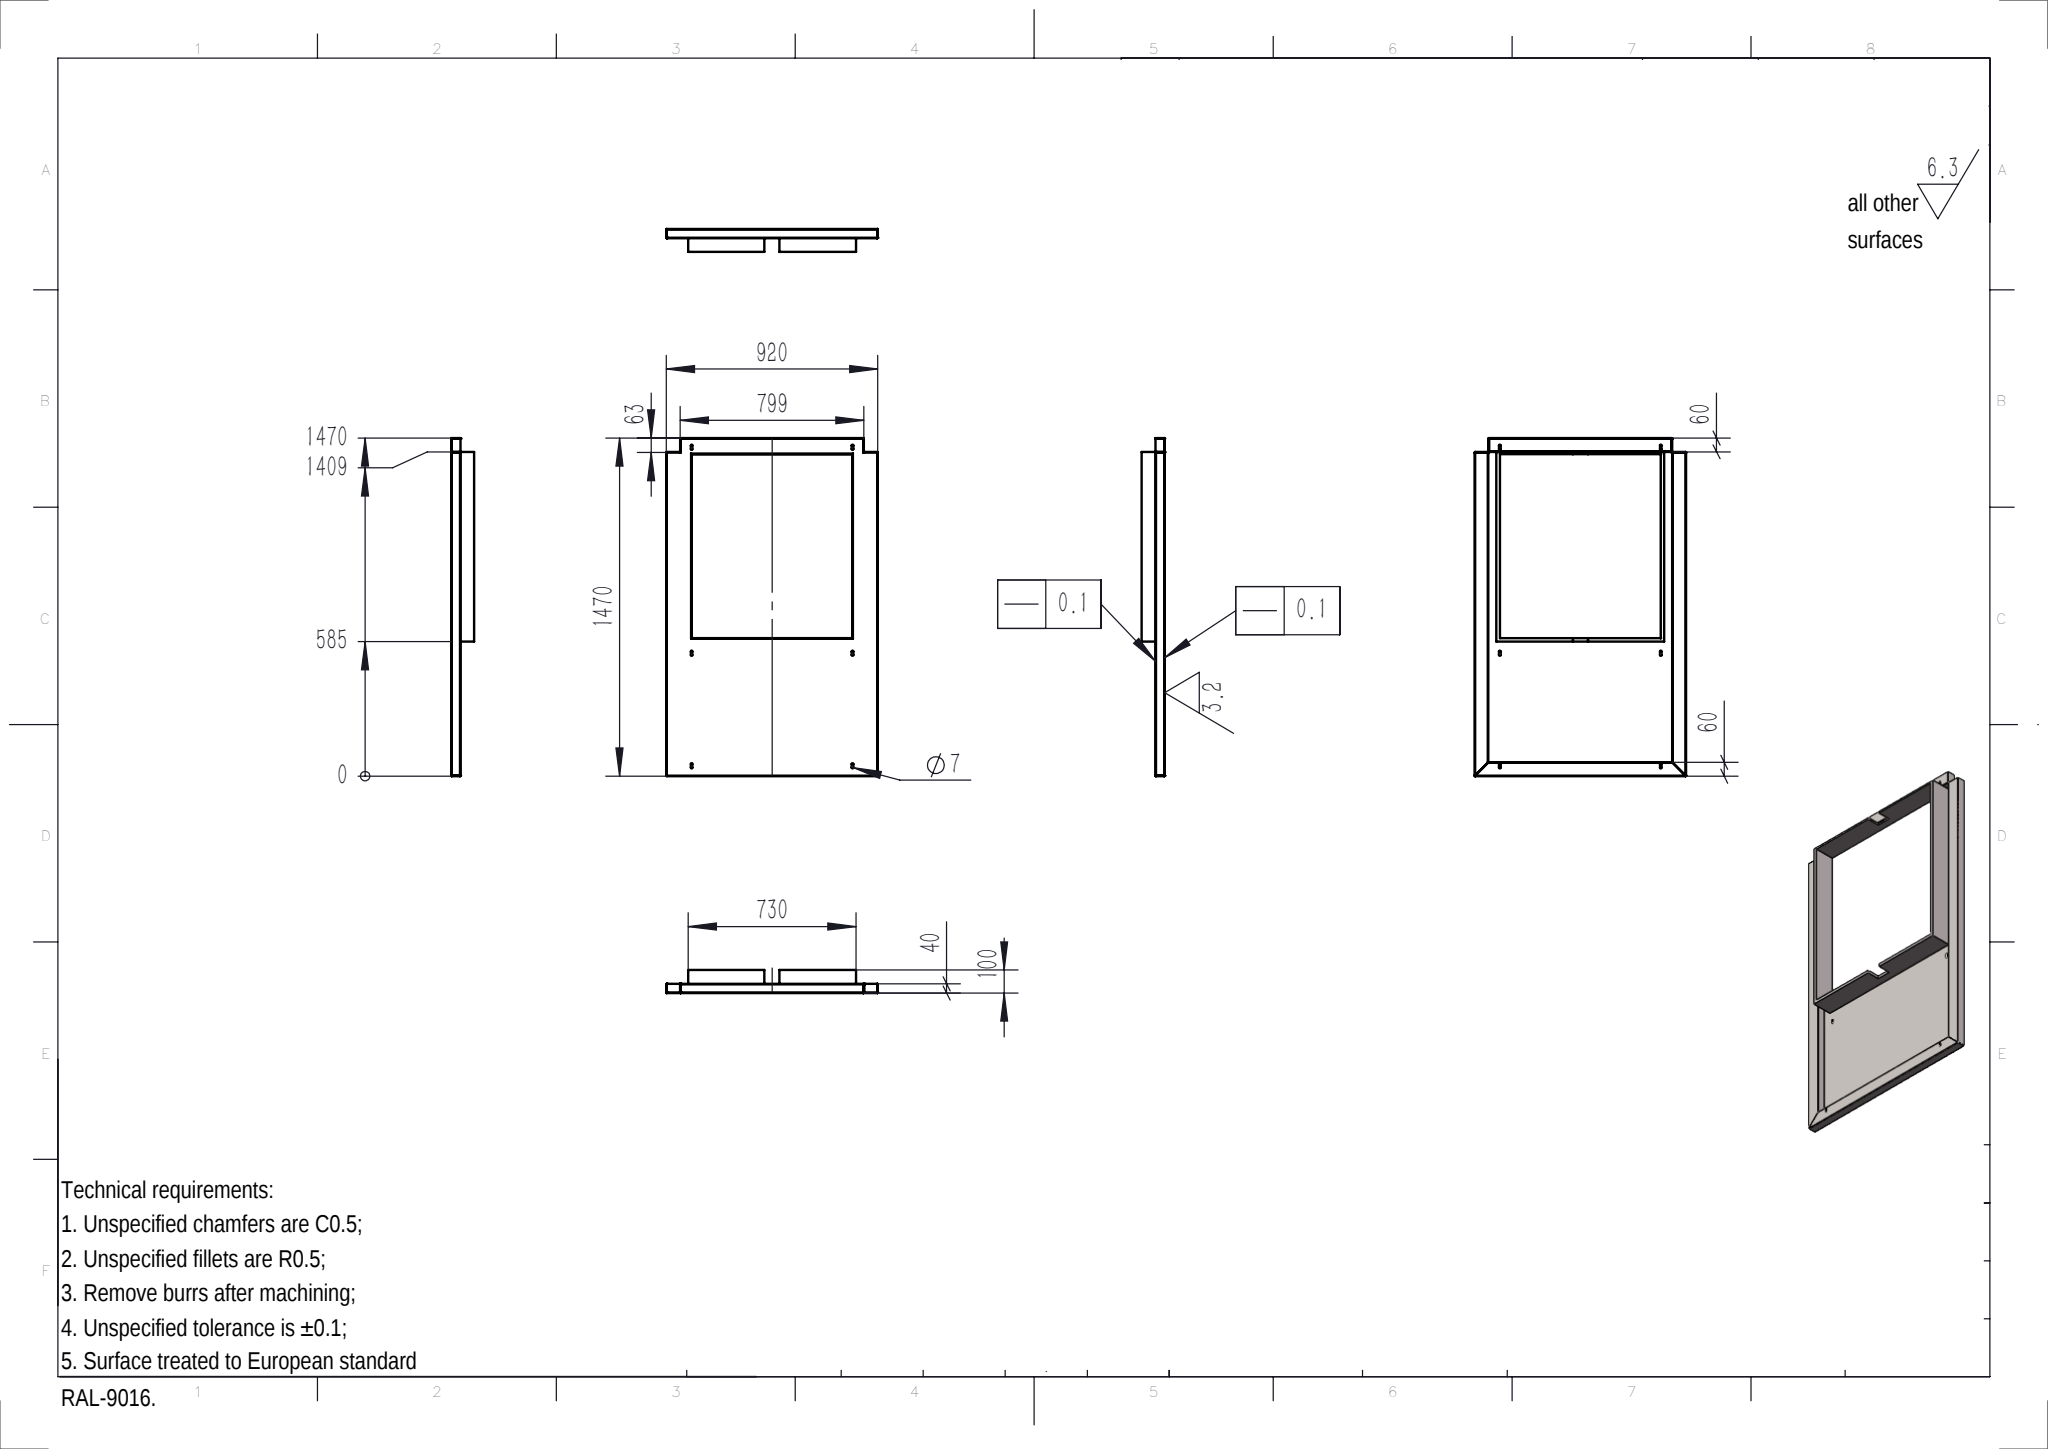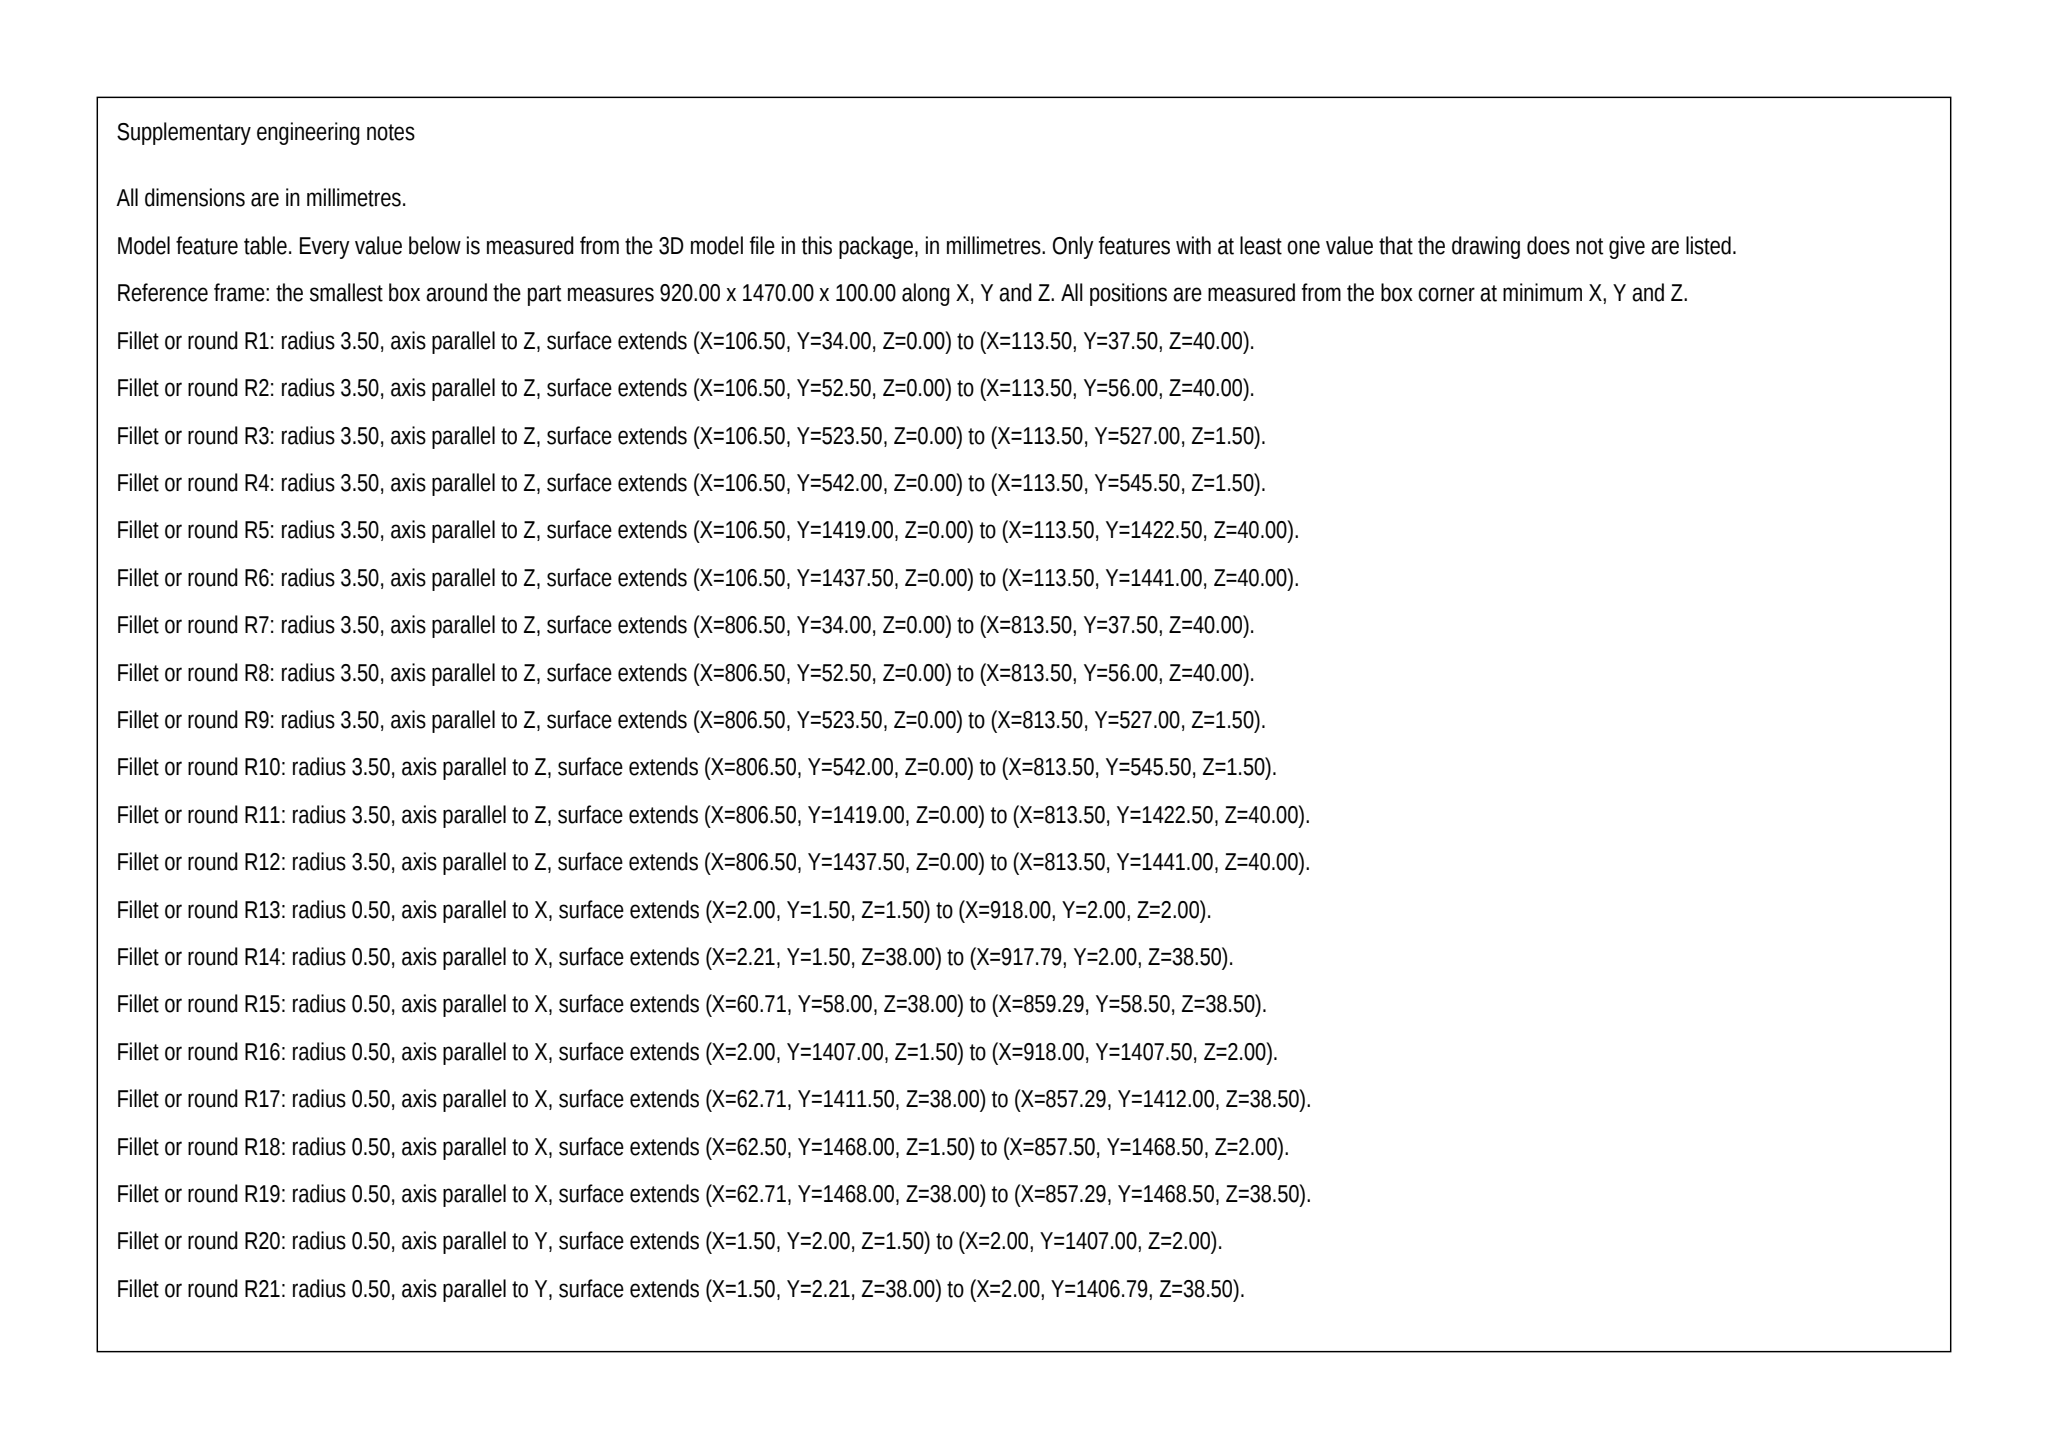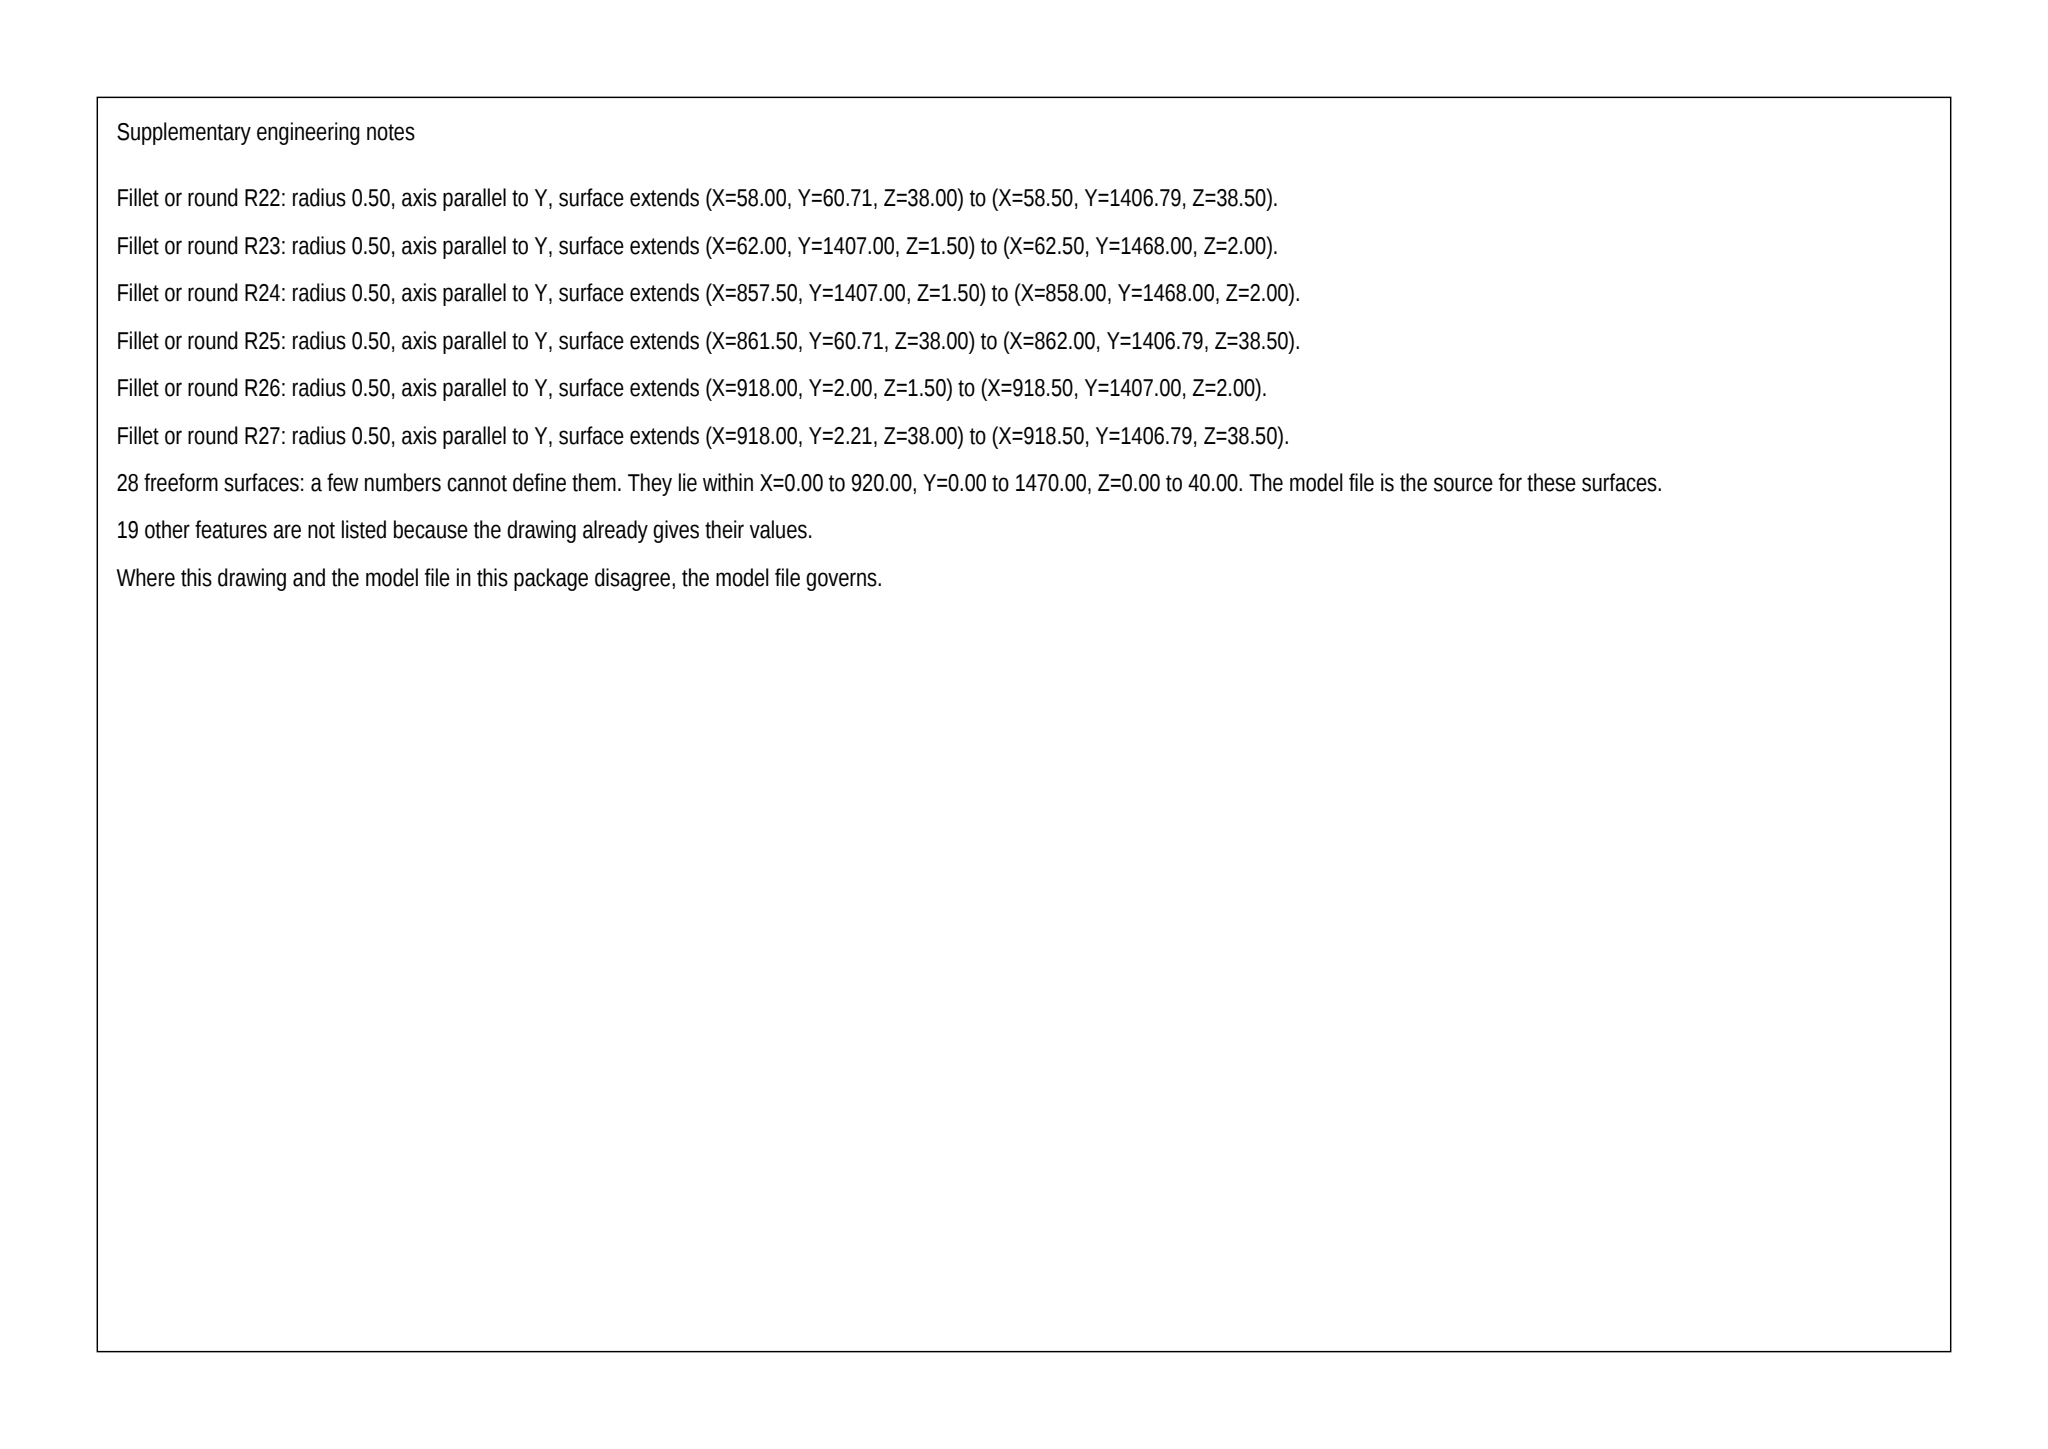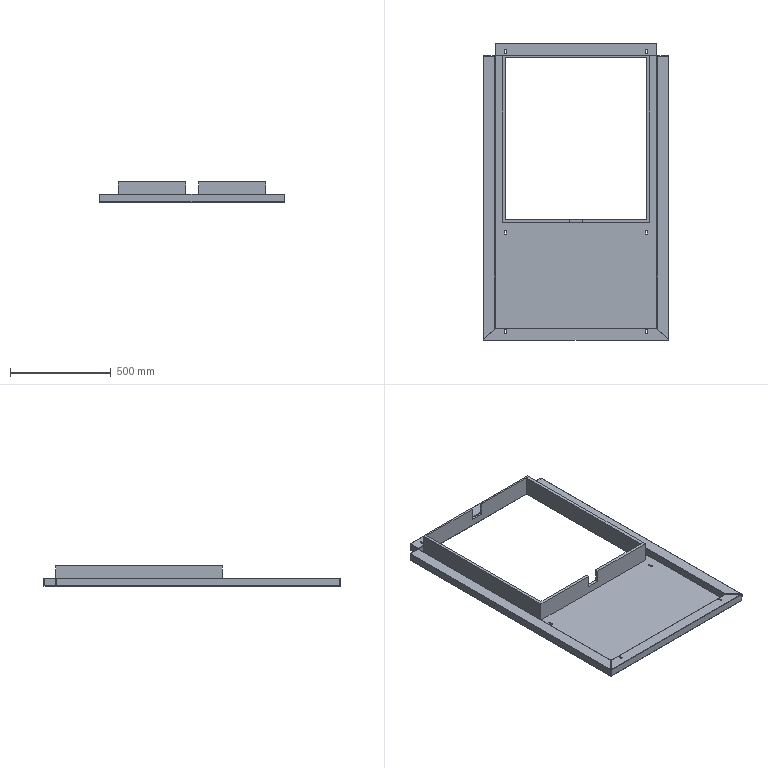Part | SolidWorks | mm | 1 solid | 215 faces | box 920 x 1470 x 100 mm | volume 6052505 mm3 | plane 131 | cylinder 56 | spline 28 | commonest cylinder face diameters 4 x20 7 x20 1 x16